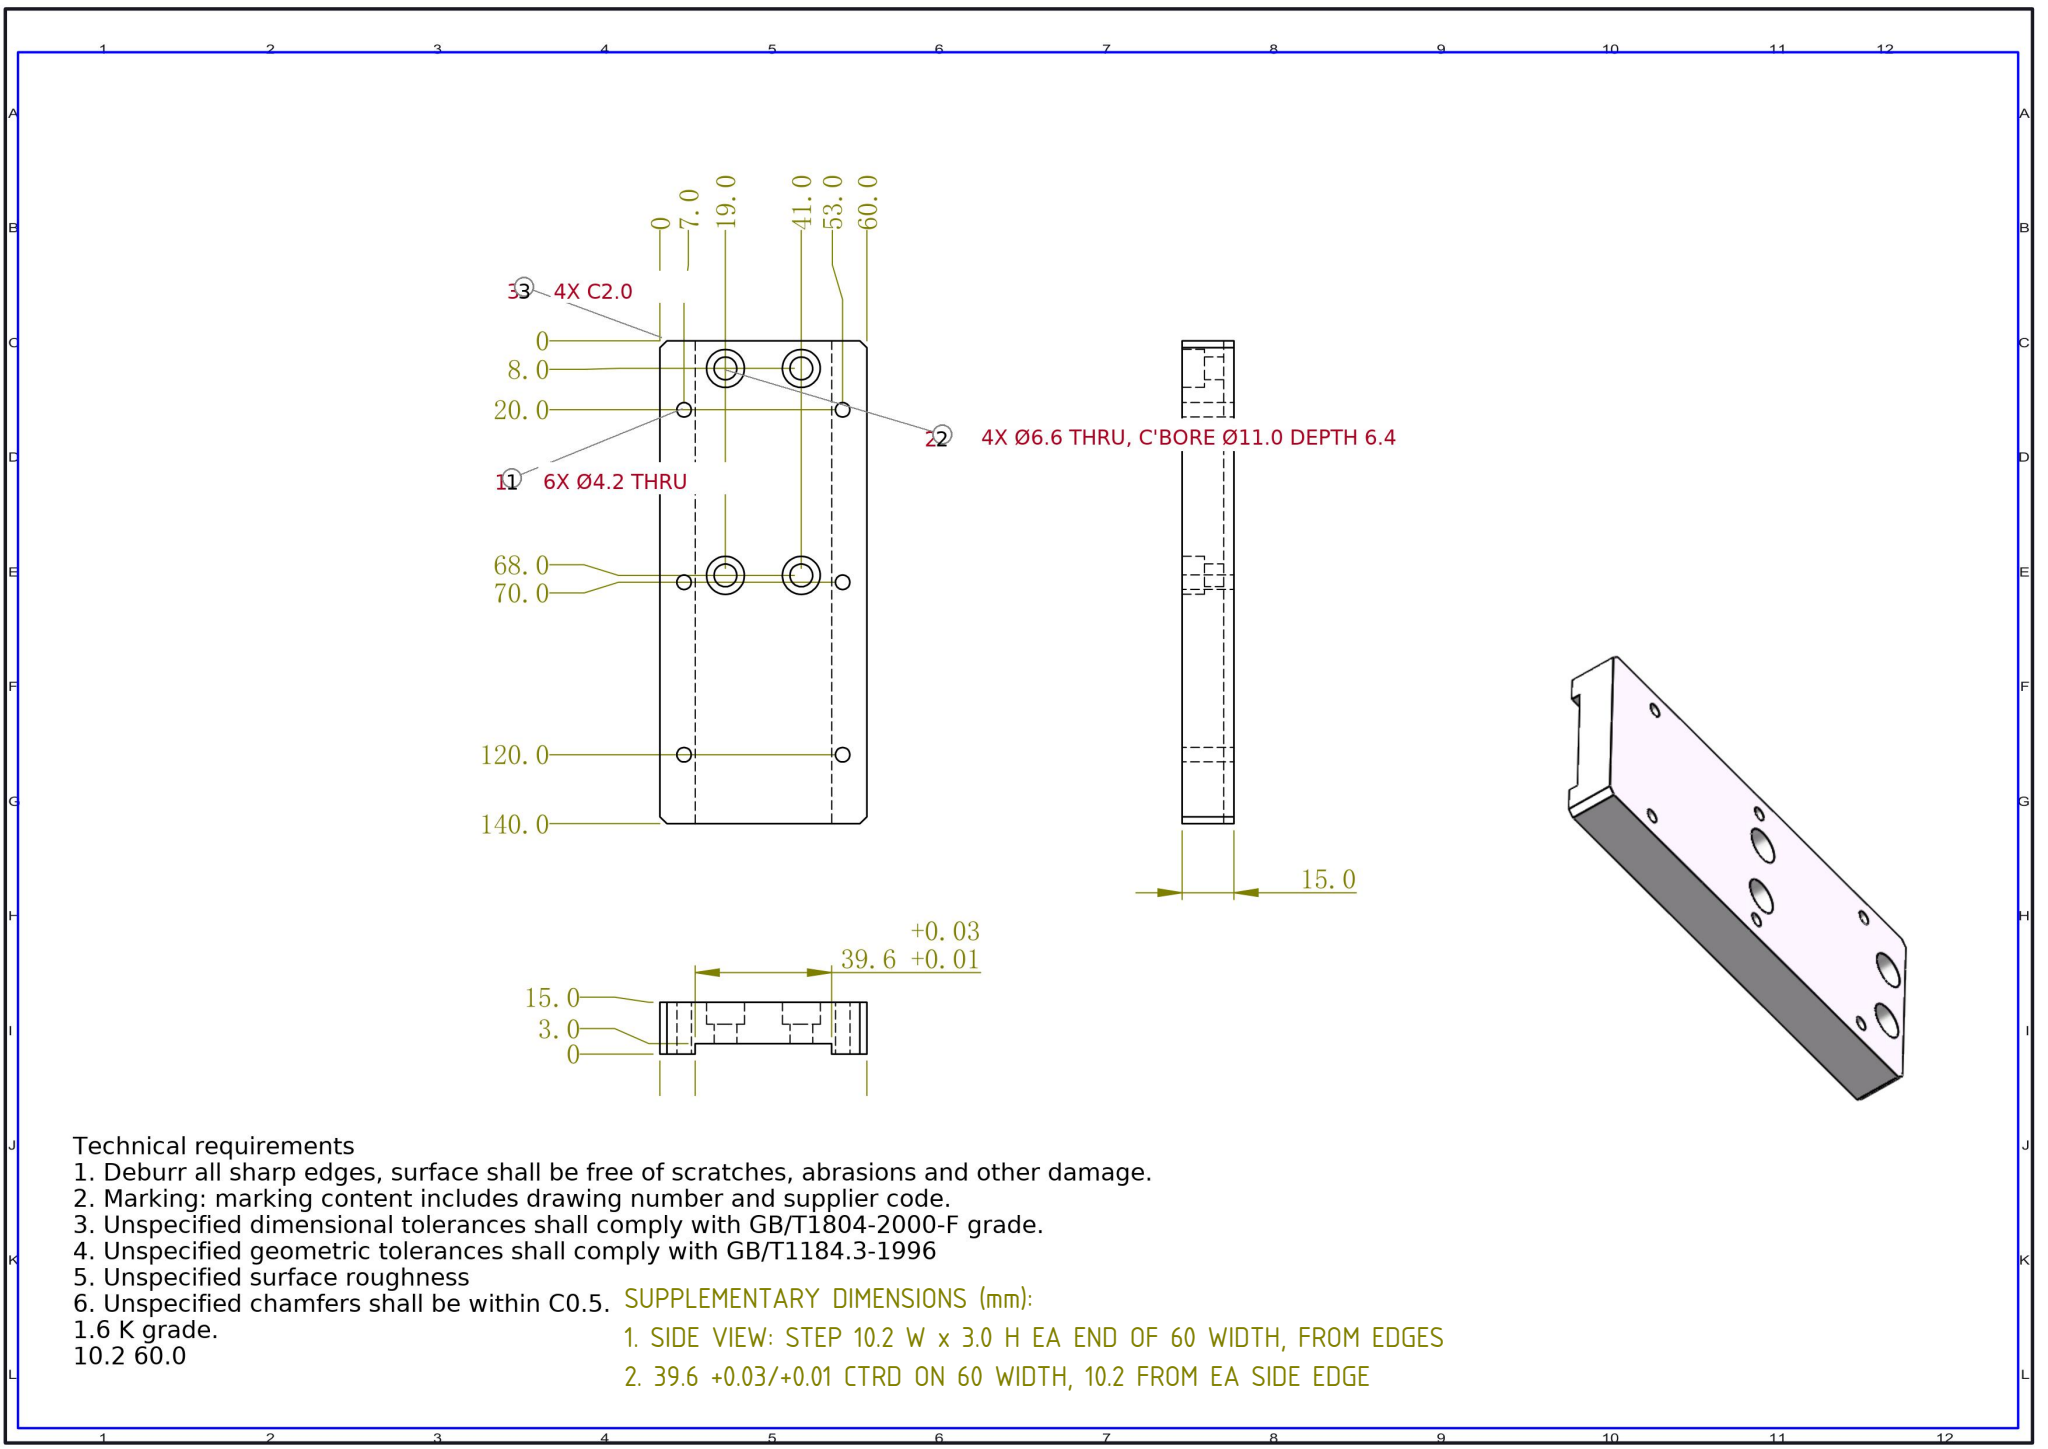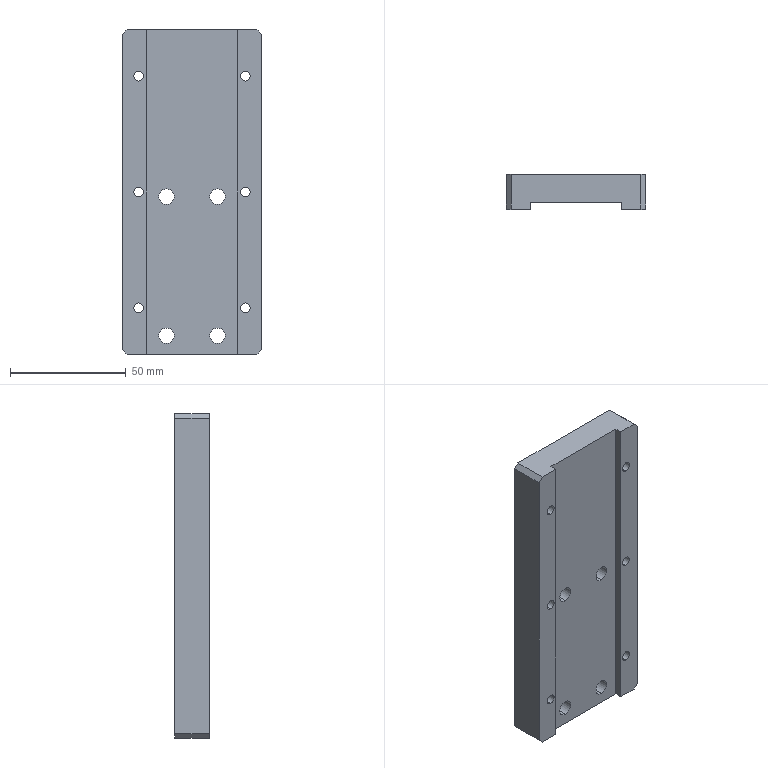Part | SolidWorks | mm | 1 solid | 46 faces | box 60 x 15 x 140 mm | volume 104802 mm3 | cylinder 28 | plane 18 | commonest cylinder face diameters 4.2 x12 11 x8 6.6 x8
build123d program:
from build123d import *

# Parameters (mm, degrees)
SKETCH1_W                                       = 60
SKETCH1_H                                       = 140
BOSS_EXTRUDE1_DEPTH                             = 15
SKETCH2_W                                       = 39.6
SKETCH2_H                                       = 140
CUT_EXTRUDE1_DEPTH                              = 3
M6_HEX_SOCKET_HEAD_CAP_SCREW_CBORE1_D           = 6.6
M6_HEX_SOCKET_HEAD_CAP_SCREW_CBORE1_CBORE_D     = 11
M6_HEX_SOCKET_HEAD_CAP_SCREW_CBORE1_CBORE_DEPTH = 6.4
M5_TAPPED_HOLE1_D                               = 4.2
CHAMFER1_SIZE                                   = 2


with BuildPart() as part:
    # Sketch1 → Boss-Extrude1 (new body)
    with BuildSketch(Plane.XZ):
        with Locations((30, 70)):
            Rectangle(SKETCH1_W, SKETCH1_H)
    extrude(amount=-BOSS_EXTRUDE1_DEPTH)

    # Sketch2 → Cut-Extrude1 (cut)
    with BuildSketch(Plane.XZ):
        with Locations((30, 70)):
            Rectangle(SKETCH2_W, SKETCH2_H)
    extrude(amount=-CUT_EXTRUDE1_DEPTH, mode=Mode.SUBTRACT)

    # M6 Hex Socket Head Cap Screw CBORE1 (through all)
    with Locations(Plane(origin=(0, 15, 0), x_dir=(1, 0, 0), z_dir=(0, 1, 0))):
        with Locations((41, -8), (19, -8), (41, -68), (19, -68)):
            CounterBoreHole(M6_HEX_SOCKET_HEAD_CAP_SCREW_CBORE1_D / 2, M6_HEX_SOCKET_HEAD_CAP_SCREW_CBORE1_CBORE_D / 2, M6_HEX_SOCKET_HEAD_CAP_SCREW_CBORE1_CBORE_DEPTH)

    # M5 Tapped Hole1 (through all)
    with Locations(Plane(origin=(0, 15, 0), x_dir=(1, 0, 0), z_dir=(0, 1, 0))):
        with Locations((7, -20), (53, -20), (7, -70), (53, -70), (53, -120), (7, -120)):
            Hole(M5_TAPPED_HOLE1_D / 2)

    # Chamfer1
    chamfer1_edges = [part.edges().sort_by_distance(p)[0] for p in [
        (60, 7.5, 140),
        (60, 7.5, 0),
        (0, 7.5, 0),
        (0, 7.5, 140),
    ]]
    chamfer(chamfer1_edges, length=CHAMFER1_SIZE)


solid = part.part